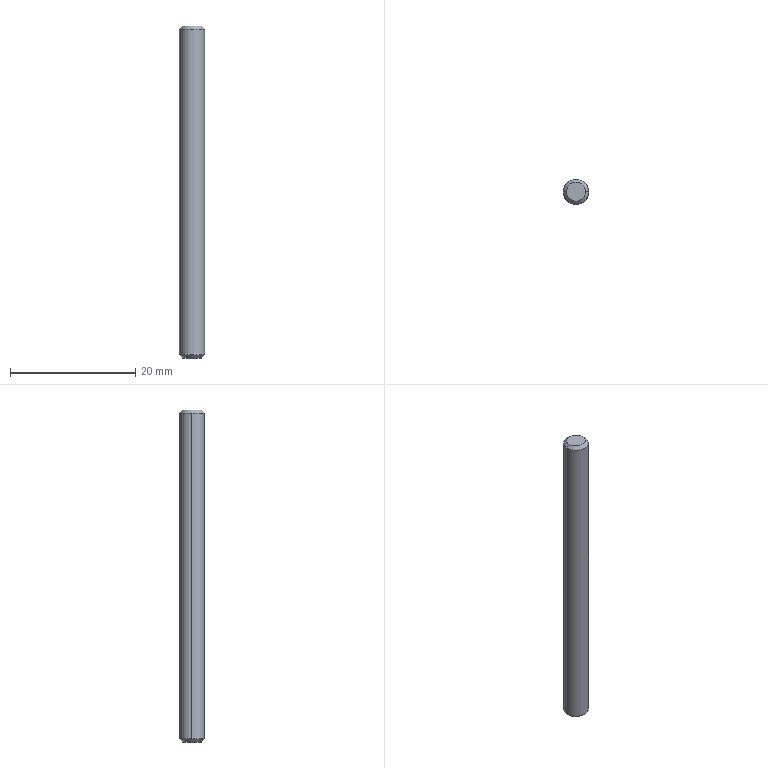Component | SolidWorks | AdhesiveRollerFixedAxis-2 | 1 solid | 8 faces | box 4 x 4 x 53 mm | volume 663 mm3 | cone 4 | cylinder 2 | plane 2 | commonest cylinder face diameters 4 x2
STEP:
#1=COLOUR_RGB('',0.7922,0.8196,0.9333);
#2=FILL_AREA_STYLE_COLOUR('',#1);
#3=FILL_AREA_STYLE('',(#2));
#4=SURFACE_STYLE_FILL_AREA(#3);
#5=SURFACE_SIDE_STYLE('',(#4));
#6=SURFACE_STYLE_USAGE(.BOTH.,#5);
#7=PRESENTATION_STYLE_ASSIGNMENT((#6));
#8=CARTESIAN_POINT('',(-6.285,3.455,0.2221));
#9=VERTEX_POINT('',#8);
#10=CARTESIAN_POINT('',(-6.443,3.455,0.2221));
#11=VERTEX_POINT('',#10);
#12=CARTESIAN_POINT('',(-6.364,3.455,0.2221));
#13=DIRECTION('',(0.,-0.,1.));
#14=DIRECTION('',(1.,-0.,0.));
#15=AXIS2_PLACEMENT_3D('',#12,#13,#14);
#16=CIRCLE('',#15,0.07874);
#17=EDGE_CURVE('',#9,#11,#16,.T.);
#18=ORIENTED_EDGE('',*,*,#17,.T.);
#19=CARTESIAN_POINT('',(-6.443,3.455,2.269));
#20=VERTEX_POINT('',#19);
#21=CARTESIAN_POINT('',(-6.443,3.455,0.2024));
#22=DIRECTION('',(0.,-0.,1.));
#23=VECTOR('',#22,39.37);
#24=LINE('',#21,#23);
#25=EDGE_CURVE('',#11,#20,#24,.T.);
#26=ORIENTED_EDGE('',*,*,#25,.T.);
#27=CARTESIAN_POINT('',(-6.285,3.455,2.269));
#28=VERTEX_POINT('',#27);
#29=CARTESIAN_POINT('',(-6.364,3.455,2.269));
#30=DIRECTION('',(-0.,0.,-1.));
#31=DIRECTION('',(1.,-0.,0.));
#32=AXIS2_PLACEMENT_3D('',#29,#30,#31);
#33=CIRCLE('',#32,0.07874);
#34=EDGE_CURVE('',#20,#28,#33,.T.);
#35=ORIENTED_EDGE('',*,*,#34,.T.);
#36=CARTESIAN_POINT('',(-6.285,3.455,0.2024));
#37=DIRECTION('',(0.,-0.,1.));
#38=VECTOR('',#37,39.37);
#39=LINE('',#36,#38);
#40=EDGE_CURVE('',#9,#28,#39,.T.);
#41=ORIENTED_EDGE('',*,*,#40,.F.);
#42=EDGE_LOOP('',(#18,#26,#35,#41));
#43=FACE_OUTER_BOUND('',#42,.T.);
#44=CARTESIAN_POINT('',(-6.364,3.455,0.2024));
#45=DIRECTION('',(0.,-0.,1.));
#46=DIRECTION('',(1.,-0.,0.));
#47=AXIS2_PLACEMENT_3D('',#44,#45,#46);
#48=CYLINDRICAL_SURFACE('',#47,0.07874);
#49=ADVANCED_FACE('',(#43),#48,.T.);
#50=CARTESIAN_POINT('',(-6.423,3.455,2.289));
#51=VERTEX_POINT('',#50);
#52=CARTESIAN_POINT('',(-6.305,3.455,2.289));
#53=VERTEX_POINT('',#52);
#54=CARTESIAN_POINT('',(-6.364,3.455,2.289));
#55=DIRECTION('',(-0.,0.,-1.));
#56=DIRECTION('',(-1.,0.,0.));
#57=AXIS2_PLACEMENT_3D('',#54,#55,#56);
#58=CIRCLE('',#57,0.05906);
#59=EDGE_CURVE('',#51,#53,#58,.T.);
#60=ORIENTED_EDGE('',*,*,#59,.T.);
#61=CARTESIAN_POINT('',(-6.285,3.455,2.269));
#62=DIRECTION('',(0.7071,-0.,-0.7071));
#63=VECTOR('',#62,39.37);
#64=LINE('',#61,#63);
#65=EDGE_CURVE('',#53,#28,#64,.T.);
#66=ORIENTED_EDGE('',*,*,#65,.T.);
#67=ORIENTED_EDGE('',*,*,#34,.F.);
#68=CARTESIAN_POINT('',(-6.443,3.455,2.269));
#69=DIRECTION('',(-0.7071,0.,-0.7071));
#70=VECTOR('',#69,39.37);
#71=LINE('',#68,#70);
#72=EDGE_CURVE('',#51,#20,#71,.T.);
#73=ORIENTED_EDGE('',*,*,#72,.F.);
#74=EDGE_LOOP('',(#60,#66,#67,#73));
#75=FACE_OUTER_BOUND('',#74,.T.);
#76=CARTESIAN_POINT('',(-6.364,3.455,2.269));
#77=DIRECTION('',(-0.,0.,-1.));
#78=DIRECTION('',(-1.,0.,0.));
#79=AXIS2_PLACEMENT_3D('',#76,#77,#78);
#80=CONICAL_SURFACE('',#79,0.07874,0.7854);
#81=ADVANCED_FACE('',(#75),#80,.T.);
#82=CARTESIAN_POINT('',(-6.305,3.455,0.2024));
#83=VERTEX_POINT('',#82);
#84=CARTESIAN_POINT('',(-6.423,3.455,0.2024));
#85=VERTEX_POINT('',#84);
#86=CARTESIAN_POINT('',(-6.364,3.455,0.2024));
#87=DIRECTION('',(0.,-0.,1.));
#88=DIRECTION('',(1.,-0.,0.));
#89=AXIS2_PLACEMENT_3D('',#86,#87,#88);
#90=CIRCLE('',#89,0.05906);
#91=EDGE_CURVE('',#83,#85,#90,.T.);
#92=ORIENTED_EDGE('',*,*,#91,.T.);
#93=CARTESIAN_POINT('',(-6.443,3.455,0.2221));
#94=DIRECTION('',(-0.7071,0.,0.7071));
#95=VECTOR('',#94,39.37);
#96=LINE('',#93,#95);
#97=EDGE_CURVE('',#85,#11,#96,.T.);
#98=ORIENTED_EDGE('',*,*,#97,.T.);
#99=ORIENTED_EDGE('',*,*,#17,.F.);
#100=CARTESIAN_POINT('',(-6.285,3.455,0.2221));
#101=DIRECTION('',(0.7071,-0.,0.7071));
#102=VECTOR('',#101,39.37);
#103=LINE('',#100,#102);
#104=EDGE_CURVE('',#83,#9,#103,.T.);
#105=ORIENTED_EDGE('',*,*,#104,.F.);
#106=EDGE_LOOP('',(#92,#98,#99,#105));
#107=FACE_OUTER_BOUND('',#106,.T.);
#108=CARTESIAN_POINT('',(-6.364,3.455,0.2221));
#109=DIRECTION('',(0.,-0.,1.));
#110=DIRECTION('',(1.,-0.,0.));
#111=AXIS2_PLACEMENT_3D('',#108,#109,#110);
#112=CONICAL_SURFACE('',#111,0.07874,0.7854);
#113=ADVANCED_FACE('',(#107),#112,.T.);
#114=ORIENTED_EDGE('',*,*,#25,.F.);
#115=CARTESIAN_POINT('',(-6.364,3.455,0.2221));
#116=DIRECTION('',(0.,-0.,1.));
#117=DIRECTION('',(1.,-0.,0.));
#118=AXIS2_PLACEMENT_3D('',#115,#116,#117);
#119=CIRCLE('',#118,0.07874);
#120=EDGE_CURVE('',#11,#9,#119,.T.);
#121=ORIENTED_EDGE('',*,*,#120,.T.);
#122=ORIENTED_EDGE('',*,*,#40,.T.);
#123=CARTESIAN_POINT('',(-6.364,3.455,2.269));
#124=DIRECTION('',(-0.,0.,-1.));
#125=DIRECTION('',(1.,-0.,0.));
#126=AXIS2_PLACEMENT_3D('',#123,#124,#125);
#127=CIRCLE('',#126,0.07874);
#128=EDGE_CURVE('',#28,#20,#127,.T.);
#129=ORIENTED_EDGE('',*,*,#128,.T.);
#130=EDGE_LOOP('',(#114,#121,#122,#129));
#131=FACE_OUTER_BOUND('',#130,.T.);
#132=CARTESIAN_POINT('',(-6.364,3.455,0.2024));
#133=DIRECTION('',(0.,-0.,1.));
#134=DIRECTION('',(1.,-0.,0.));
#135=AXIS2_PLACEMENT_3D('',#132,#133,#134);
#136=CYLINDRICAL_SURFACE('',#135,0.07874);
#137=ADVANCED_FACE('',(#131),#136,.T.);
#138=ORIENTED_EDGE('',*,*,#65,.F.);
#139=CARTESIAN_POINT('',(-6.364,3.455,2.289));
#140=DIRECTION('',(-0.,0.,-1.));
#141=DIRECTION('',(-1.,0.,0.));
#142=AXIS2_PLACEMENT_3D('',#139,#140,#141);
#143=CIRCLE('',#142,0.05906);
#144=EDGE_CURVE('',#53,#51,#143,.T.);
#145=ORIENTED_EDGE('',*,*,#144,.T.);
#146=ORIENTED_EDGE('',*,*,#72,.T.);
#147=ORIENTED_EDGE('',*,*,#128,.F.);
#148=EDGE_LOOP('',(#138,#145,#146,#147));
#149=FACE_OUTER_BOUND('',#148,.T.);
#150=CARTESIAN_POINT('',(-6.364,3.455,2.269));
#151=DIRECTION('',(-0.,0.,-1.));
#152=DIRECTION('',(-1.,0.,0.));
#153=AXIS2_PLACEMENT_3D('',#150,#151,#152);
#154=CONICAL_SURFACE('',#153,0.07874,0.7854);
#155=ADVANCED_FACE('',(#149),#154,.T.);
#156=ORIENTED_EDGE('',*,*,#97,.F.);
#157=CARTESIAN_POINT('',(-6.364,3.455,0.2024));
#158=DIRECTION('',(0.,-0.,1.));
#159=DIRECTION('',(1.,-0.,0.));
#160=AXIS2_PLACEMENT_3D('',#157,#158,#159);
#161=CIRCLE('',#160,0.05906);
#162=EDGE_CURVE('',#85,#83,#161,.T.);
#163=ORIENTED_EDGE('',*,*,#162,.T.);
#164=ORIENTED_EDGE('',*,*,#104,.T.);
#165=ORIENTED_EDGE('',*,*,#120,.F.);
#166=EDGE_LOOP('',(#156,#163,#164,#165));
#167=FACE_OUTER_BOUND('',#166,.T.);
#168=CARTESIAN_POINT('',(-6.364,3.455,0.2221));
#169=DIRECTION('',(0.,-0.,1.));
#170=DIRECTION('',(1.,-0.,0.));
#171=AXIS2_PLACEMENT_3D('',#168,#169,#170);
#172=CONICAL_SURFACE('',#171,0.07874,0.7854);
#173=ADVANCED_FACE('',(#167),#172,.T.);
#174=ORIENTED_EDGE('',*,*,#59,.F.);
#175=ORIENTED_EDGE('',*,*,#144,.F.);
#176=EDGE_LOOP('',(#174,#175));
#177=FACE_OUTER_BOUND('',#176,.T.);
#178=CARTESIAN_POINT('',(-6.364,3.455,2.289));
#179=DIRECTION('',(-0.,0.,-1.));
#180=DIRECTION('',(-1.,0.,0.));
#181=AXIS2_PLACEMENT_3D('',#178,#179,#180);
#182=PLANE('',#181);
#183=ADVANCED_FACE('',(#177),#182,.F.);
#184=ORIENTED_EDGE('',*,*,#91,.F.);
#185=ORIENTED_EDGE('',*,*,#162,.F.);
#186=EDGE_LOOP('',(#184,#185));
#187=FACE_OUTER_BOUND('',#186,.T.);
#188=CARTESIAN_POINT('',(-6.364,3.455,0.2024));
#189=DIRECTION('',(-0.,0.,-1.));
#190=DIRECTION('',(-1.,0.,0.));
#191=AXIS2_PLACEMENT_3D('',#188,#189,#190);
#192=PLANE('',#191);
#193=ADVANCED_FACE('',(#187),#192,.T.);
#194=CLOSED_SHELL('',(#49,#81,#113,#137,#155,#173,#183,#193));
#195=MANIFOLD_SOLID_BREP('',#194);
#196=STYLED_ITEM('',(#7),#195);
#197=(LENGTH_UNIT()NAMED_UNIT(*)SI_UNIT($,.METRE.));
#198=LENGTH_MEASURE_WITH_UNIT(LENGTH_MEASURE(0.0254),#197);
#199=DIMENSIONAL_EXPONENTS(1.,0.,0.,0.,0.,0.,0.);
#200=(CONVERSION_BASED_UNIT('',#198)LENGTH_UNIT()NAMED_UNIT(#199));
#201=UNCERTAINTY_MEASURE_WITH_UNIT(LENGTH_MEASURE(0.00001),#200,'','');
#202=(NAMED_UNIT(*)PLANE_ANGLE_UNIT()SI_UNIT($,.RADIAN.));
#203=(NAMED_UNIT(*)SI_UNIT($,.STERADIAN.)SOLID_ANGLE_UNIT());
#204=(GEOMETRIC_REPRESENTATION_CONTEXT(3)GLOBAL_UNCERTAINTY_ASSIGNED_CONTEXT((#201))GLOBAL_UNIT_ASSIGNED_CONTEXT((#200,#202,#203))REPRESENTATION_CONTEXT('',''));
#205=MECHANICAL_DESIGN_GEOMETRIC_PRESENTATION_REPRESENTATION('',(#196),#204);
#206=CARTESIAN_POINT('',(0.,0.,0.));
#207=DIRECTION('',(0.,0.,1.));
#208=DIRECTION('',(1.,0.,0.));
#209=AXIS2_PLACEMENT_3D('',#206,#207,#208);
#210=(LENGTH_UNIT()NAMED_UNIT(*)SI_UNIT($,.METRE.));
#211=LENGTH_MEASURE_WITH_UNIT(LENGTH_MEASURE(0.0254),#210);
#212=DIMENSIONAL_EXPONENTS(1.,0.,0.,0.,0.,0.,0.);
#213=(CONVERSION_BASED_UNIT('',#211)LENGTH_UNIT()NAMED_UNIT(#212));
#214=UNCERTAINTY_MEASURE_WITH_UNIT(LENGTH_MEASURE(0.00001),#213,'','');
#215=(NAMED_UNIT(*)PLANE_ANGLE_UNIT()SI_UNIT($,.RADIAN.));
#216=(NAMED_UNIT(*)SI_UNIT($,.STERADIAN.)SOLID_ANGLE_UNIT());
#217=(GEOMETRIC_REPRESENTATION_CONTEXT(3)GLOBAL_UNCERTAINTY_ASSIGNED_CONTEXT((#214))GLOBAL_UNIT_ASSIGNED_CONTEXT((#213,#215,#216))REPRESENTATION_CONTEXT('',''));
#218=ADVANCED_BREP_SHAPE_REPRESENTATION('',(#195,#209),#217);
#219=PRESENTATION_LAYER_ASSIGNMENT('','',(#196));